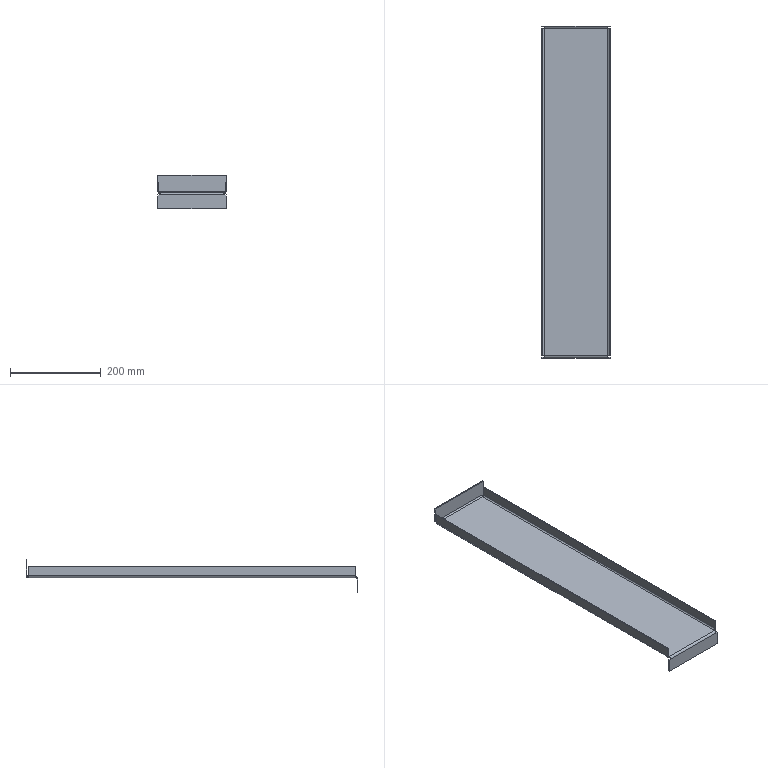Component | NX | COLUMN_LEFT_FRONT | 1 solid | 38 faces | volume 300314 mm3 | plane 30 | cylinder 8 | commonest cylinder face diameters 10 x4 6 x4